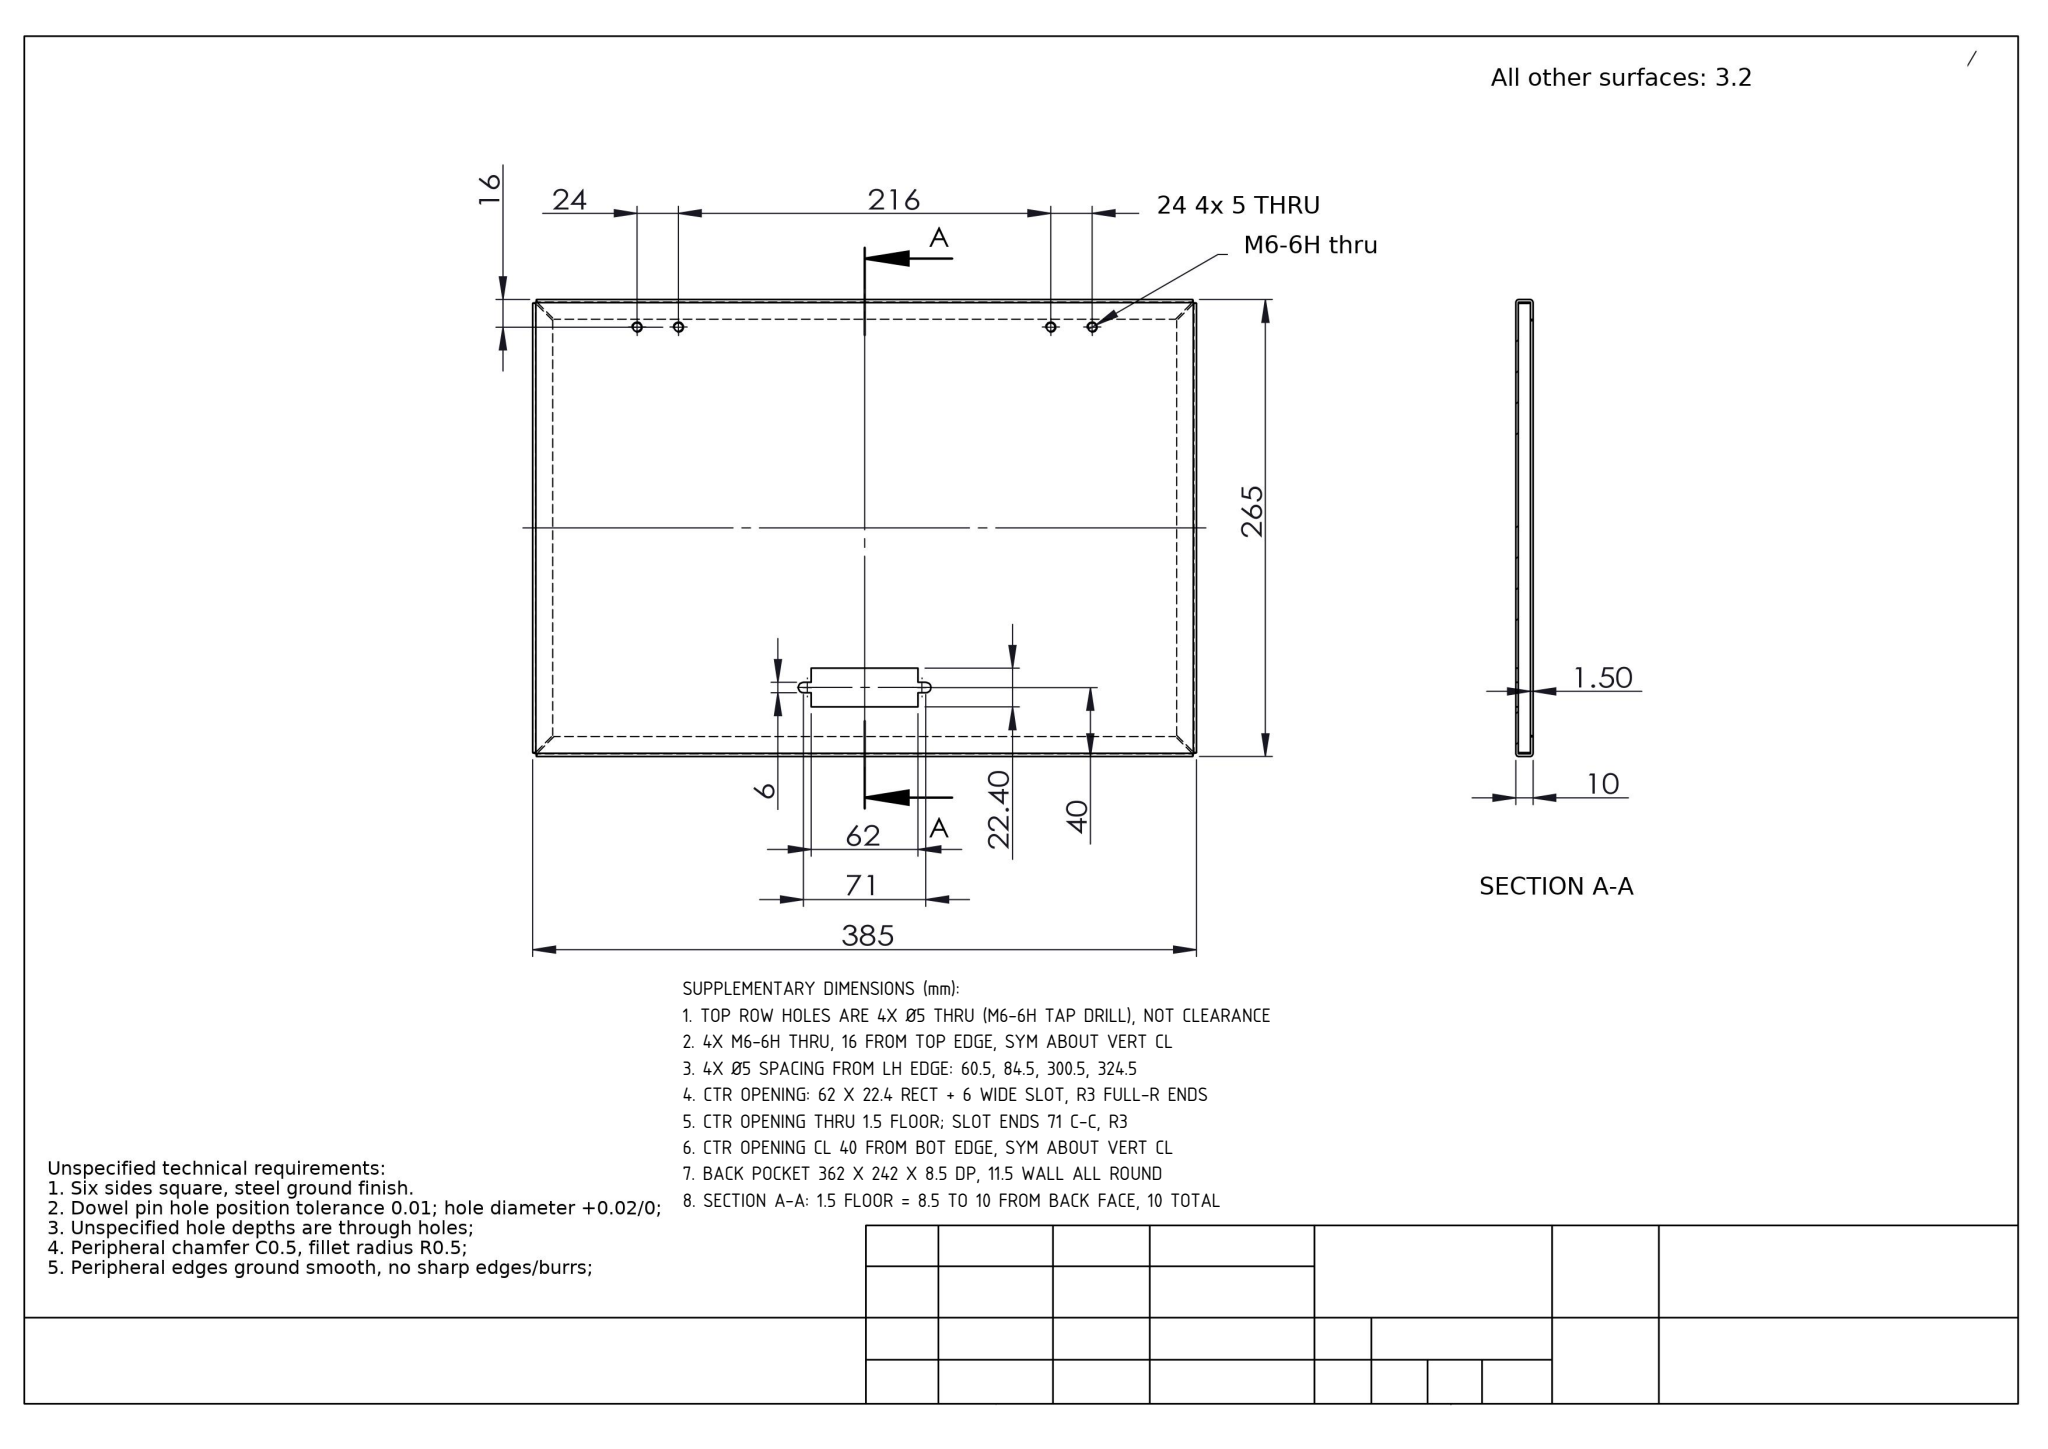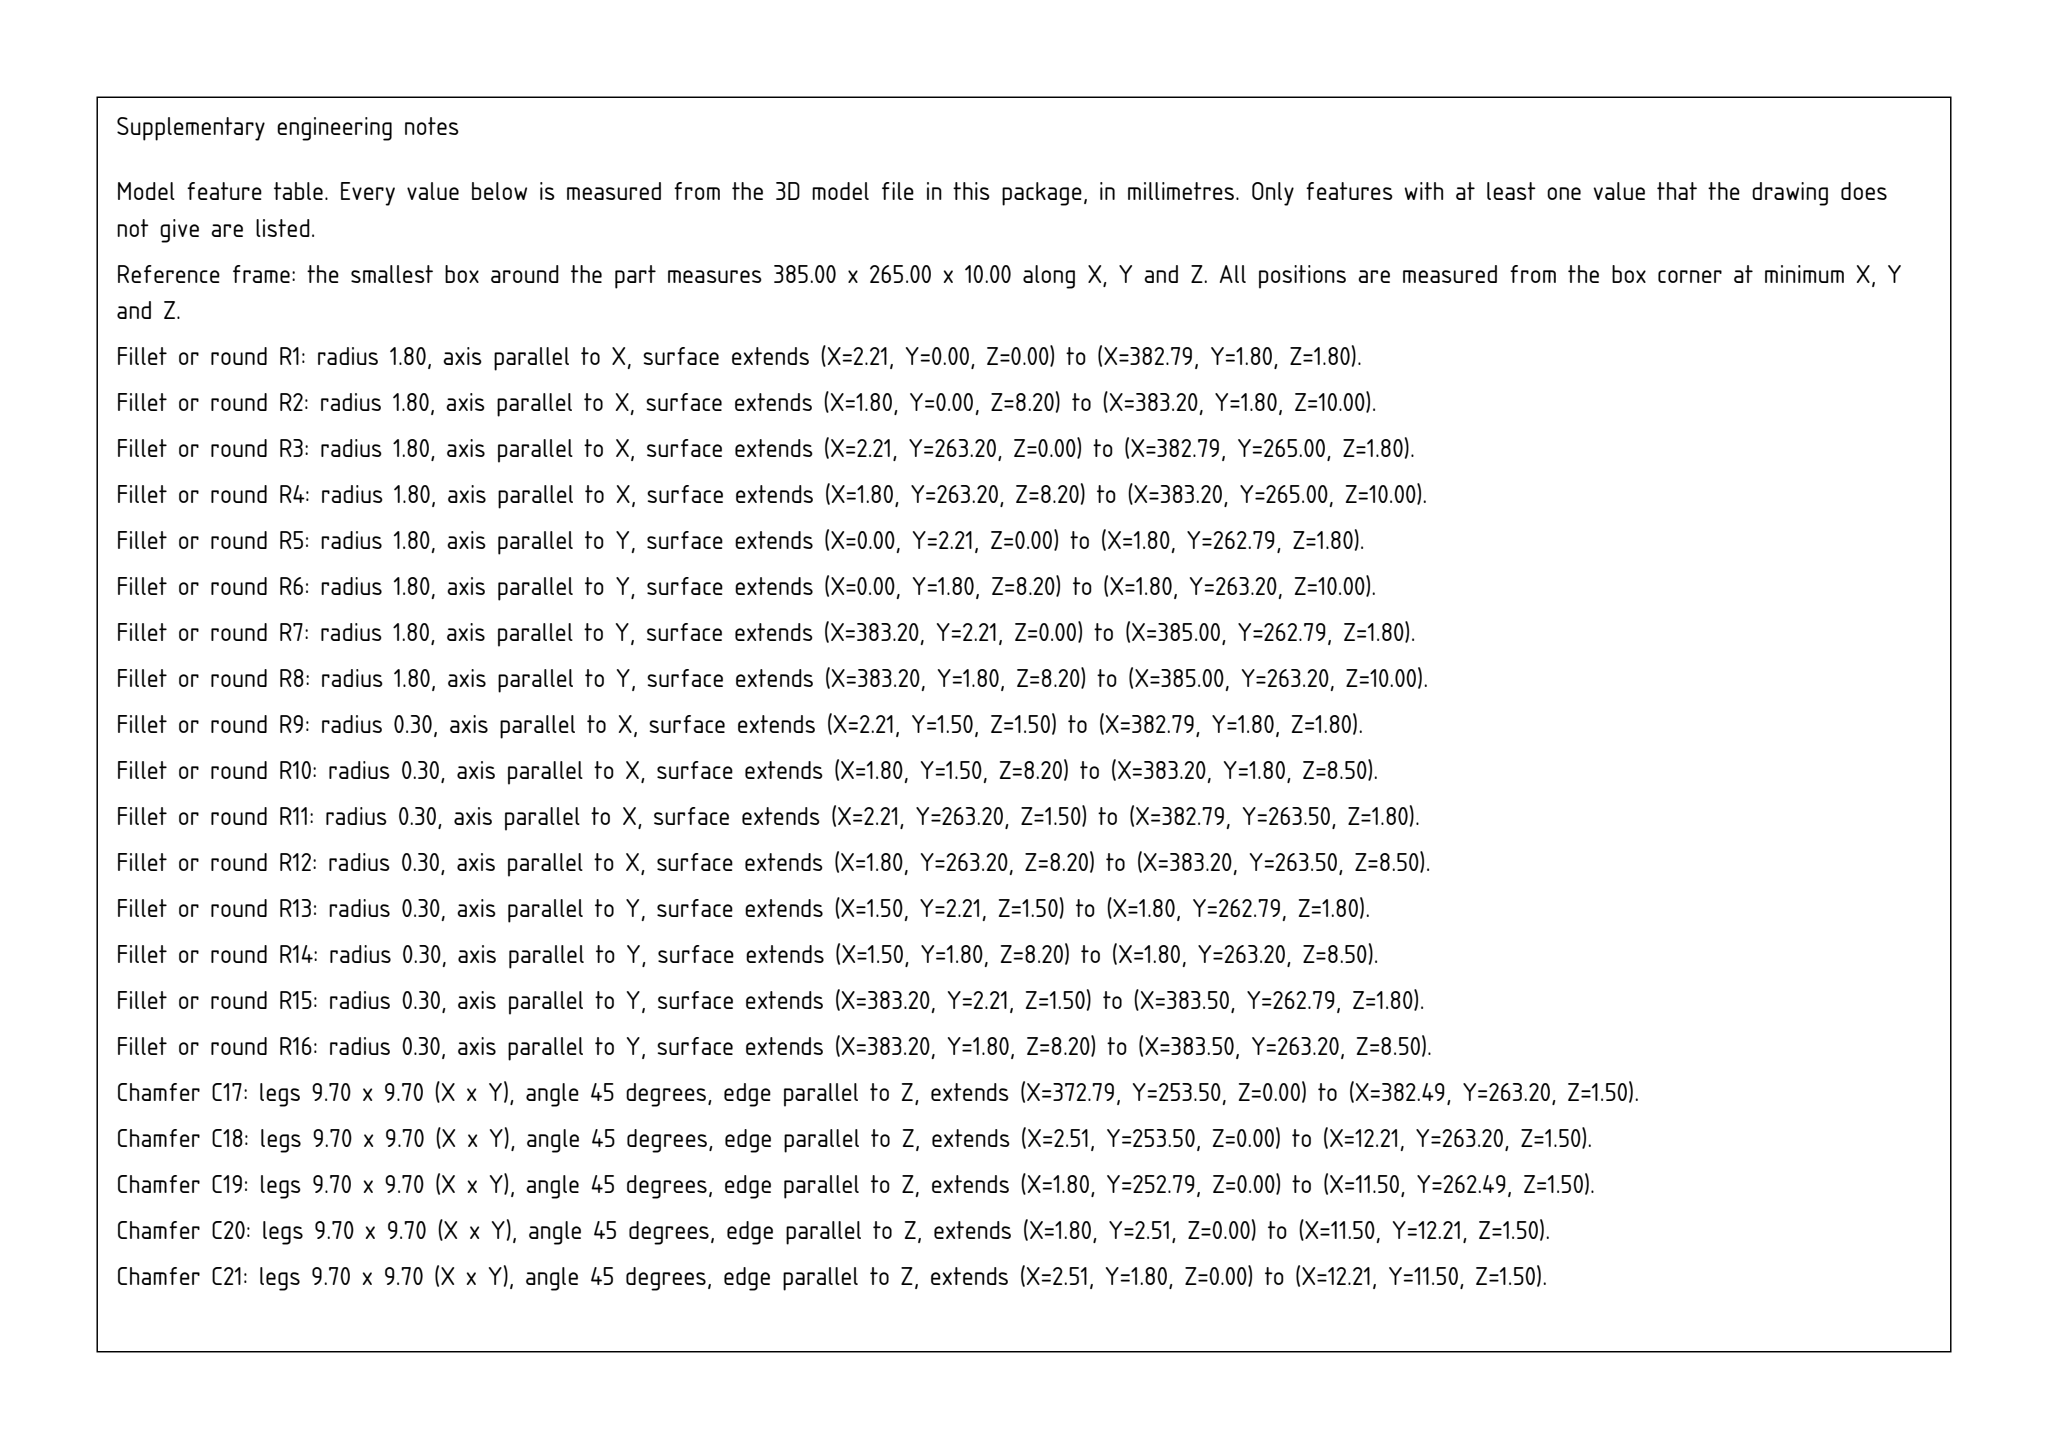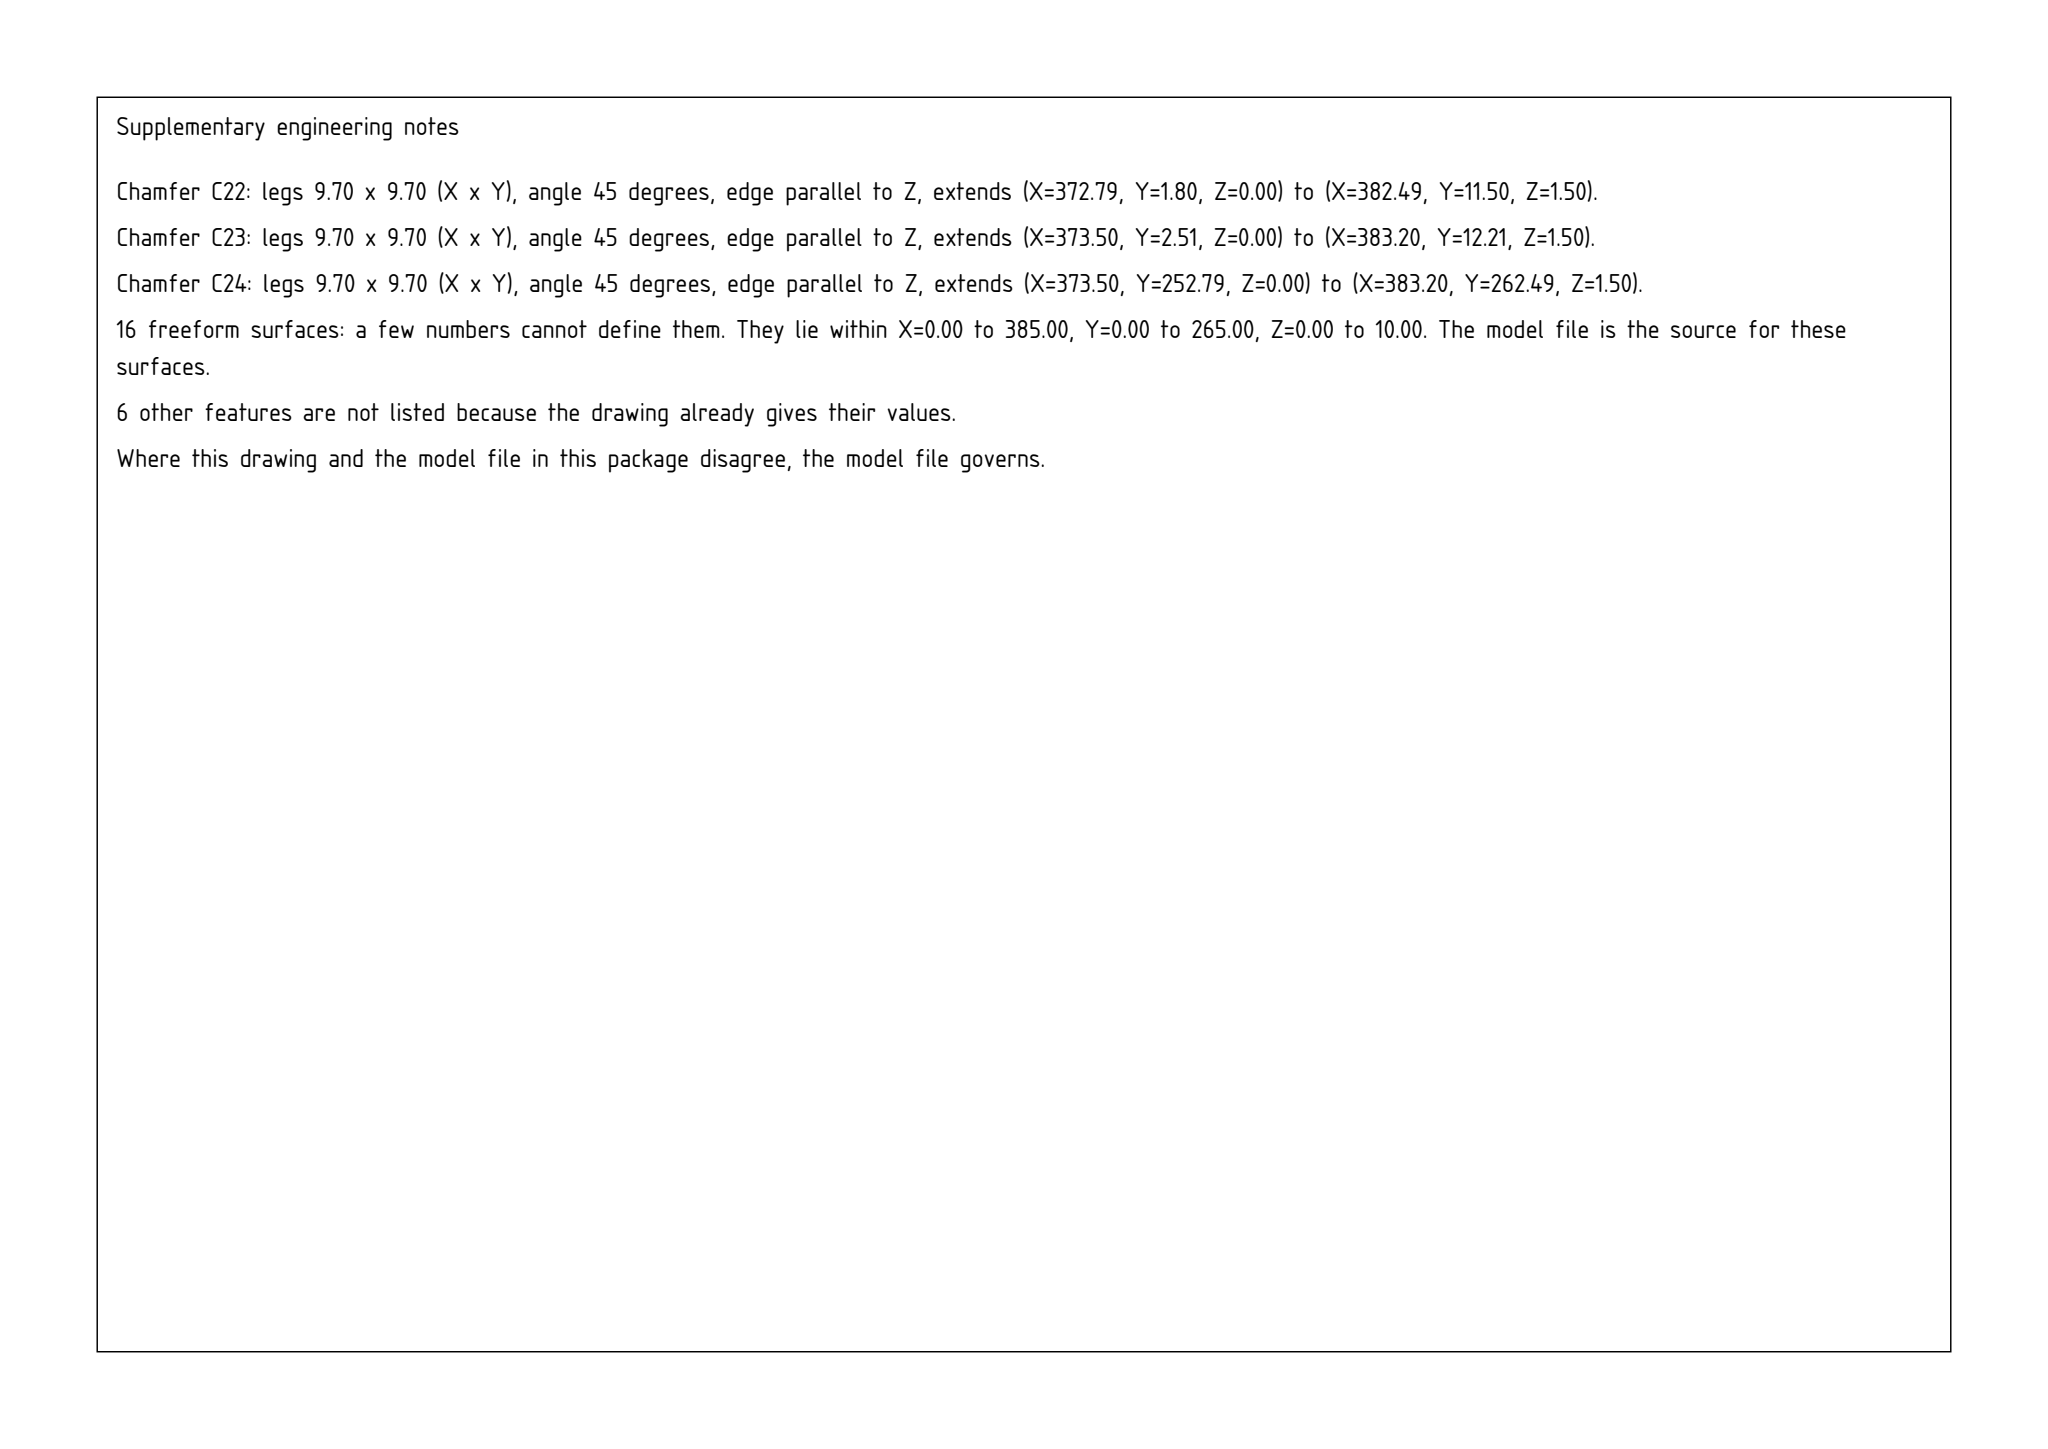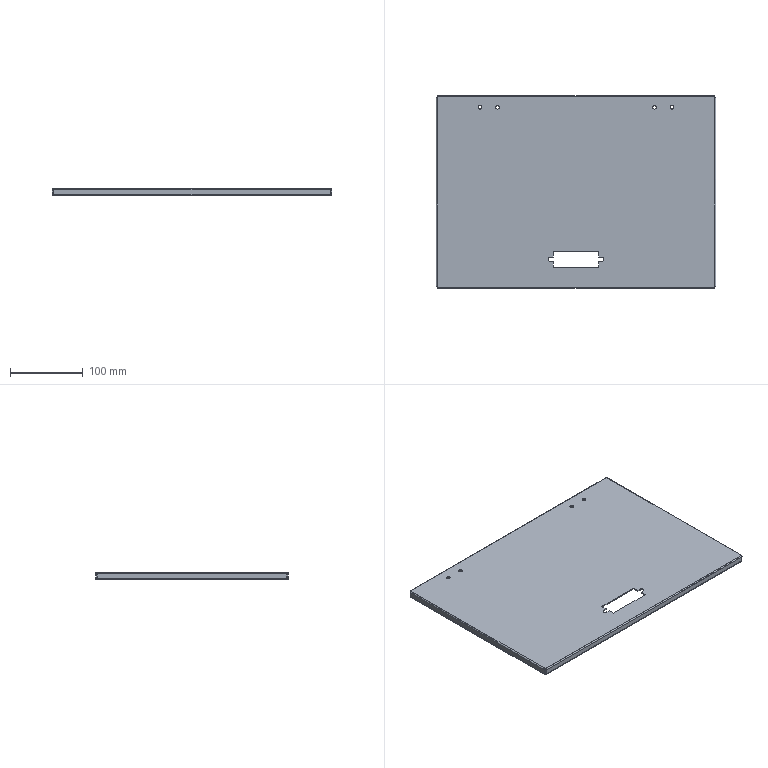Part | SolidWorks | mm | 1 solid | 91 faces | box 385 x 265 x 10 mm | volume 183938 mm3 | plane 48 | cylinder 27 | spline 16 | commonest cylinder face diameters 5 x8 3.6 x8 0.6 x8 6 x3